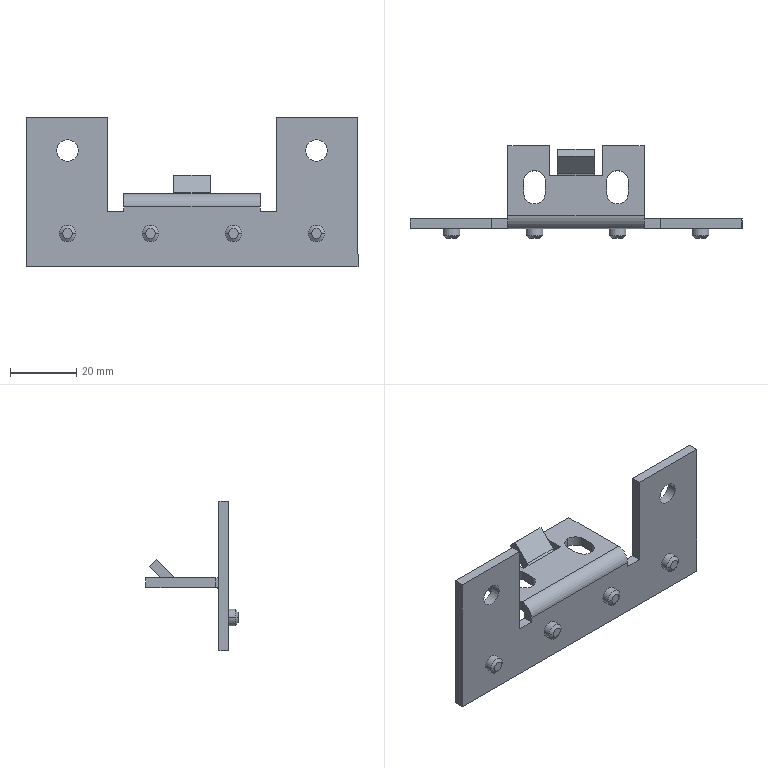Component | SolidWorks | Bracket(Item49)-4 | 1 solid | 90 faces | volume 11802 mm3 | plane 44 | cone 24 | cylinder 22 | commonest cylinder face diameters 6.5 x10 5 x8 8 x2 2 x2 | material Plain Carbon Steel